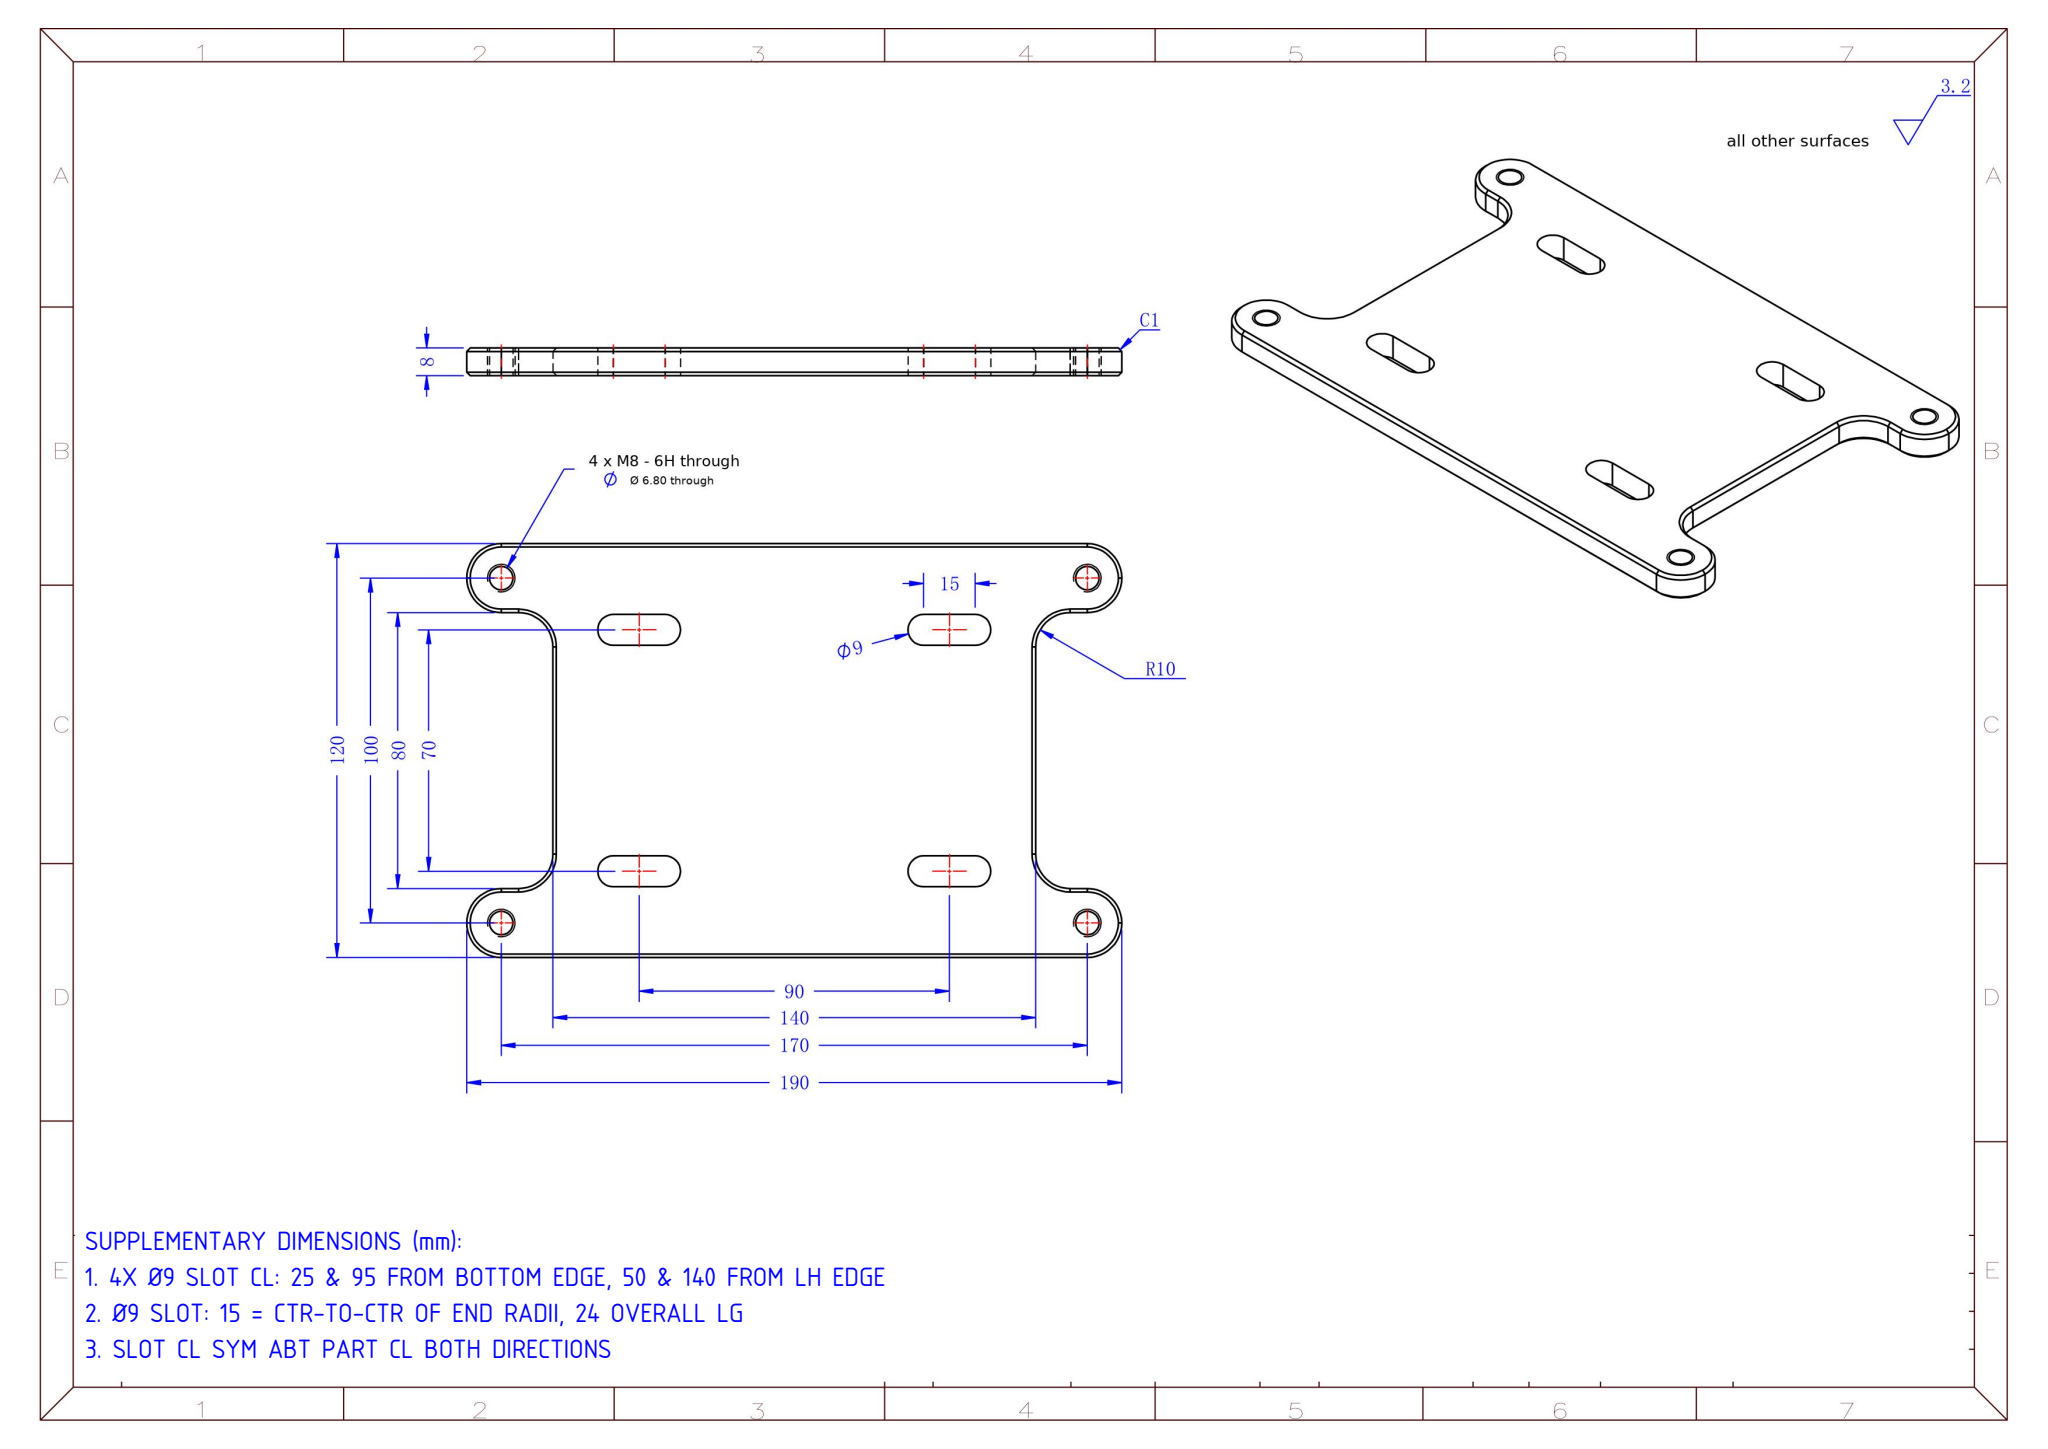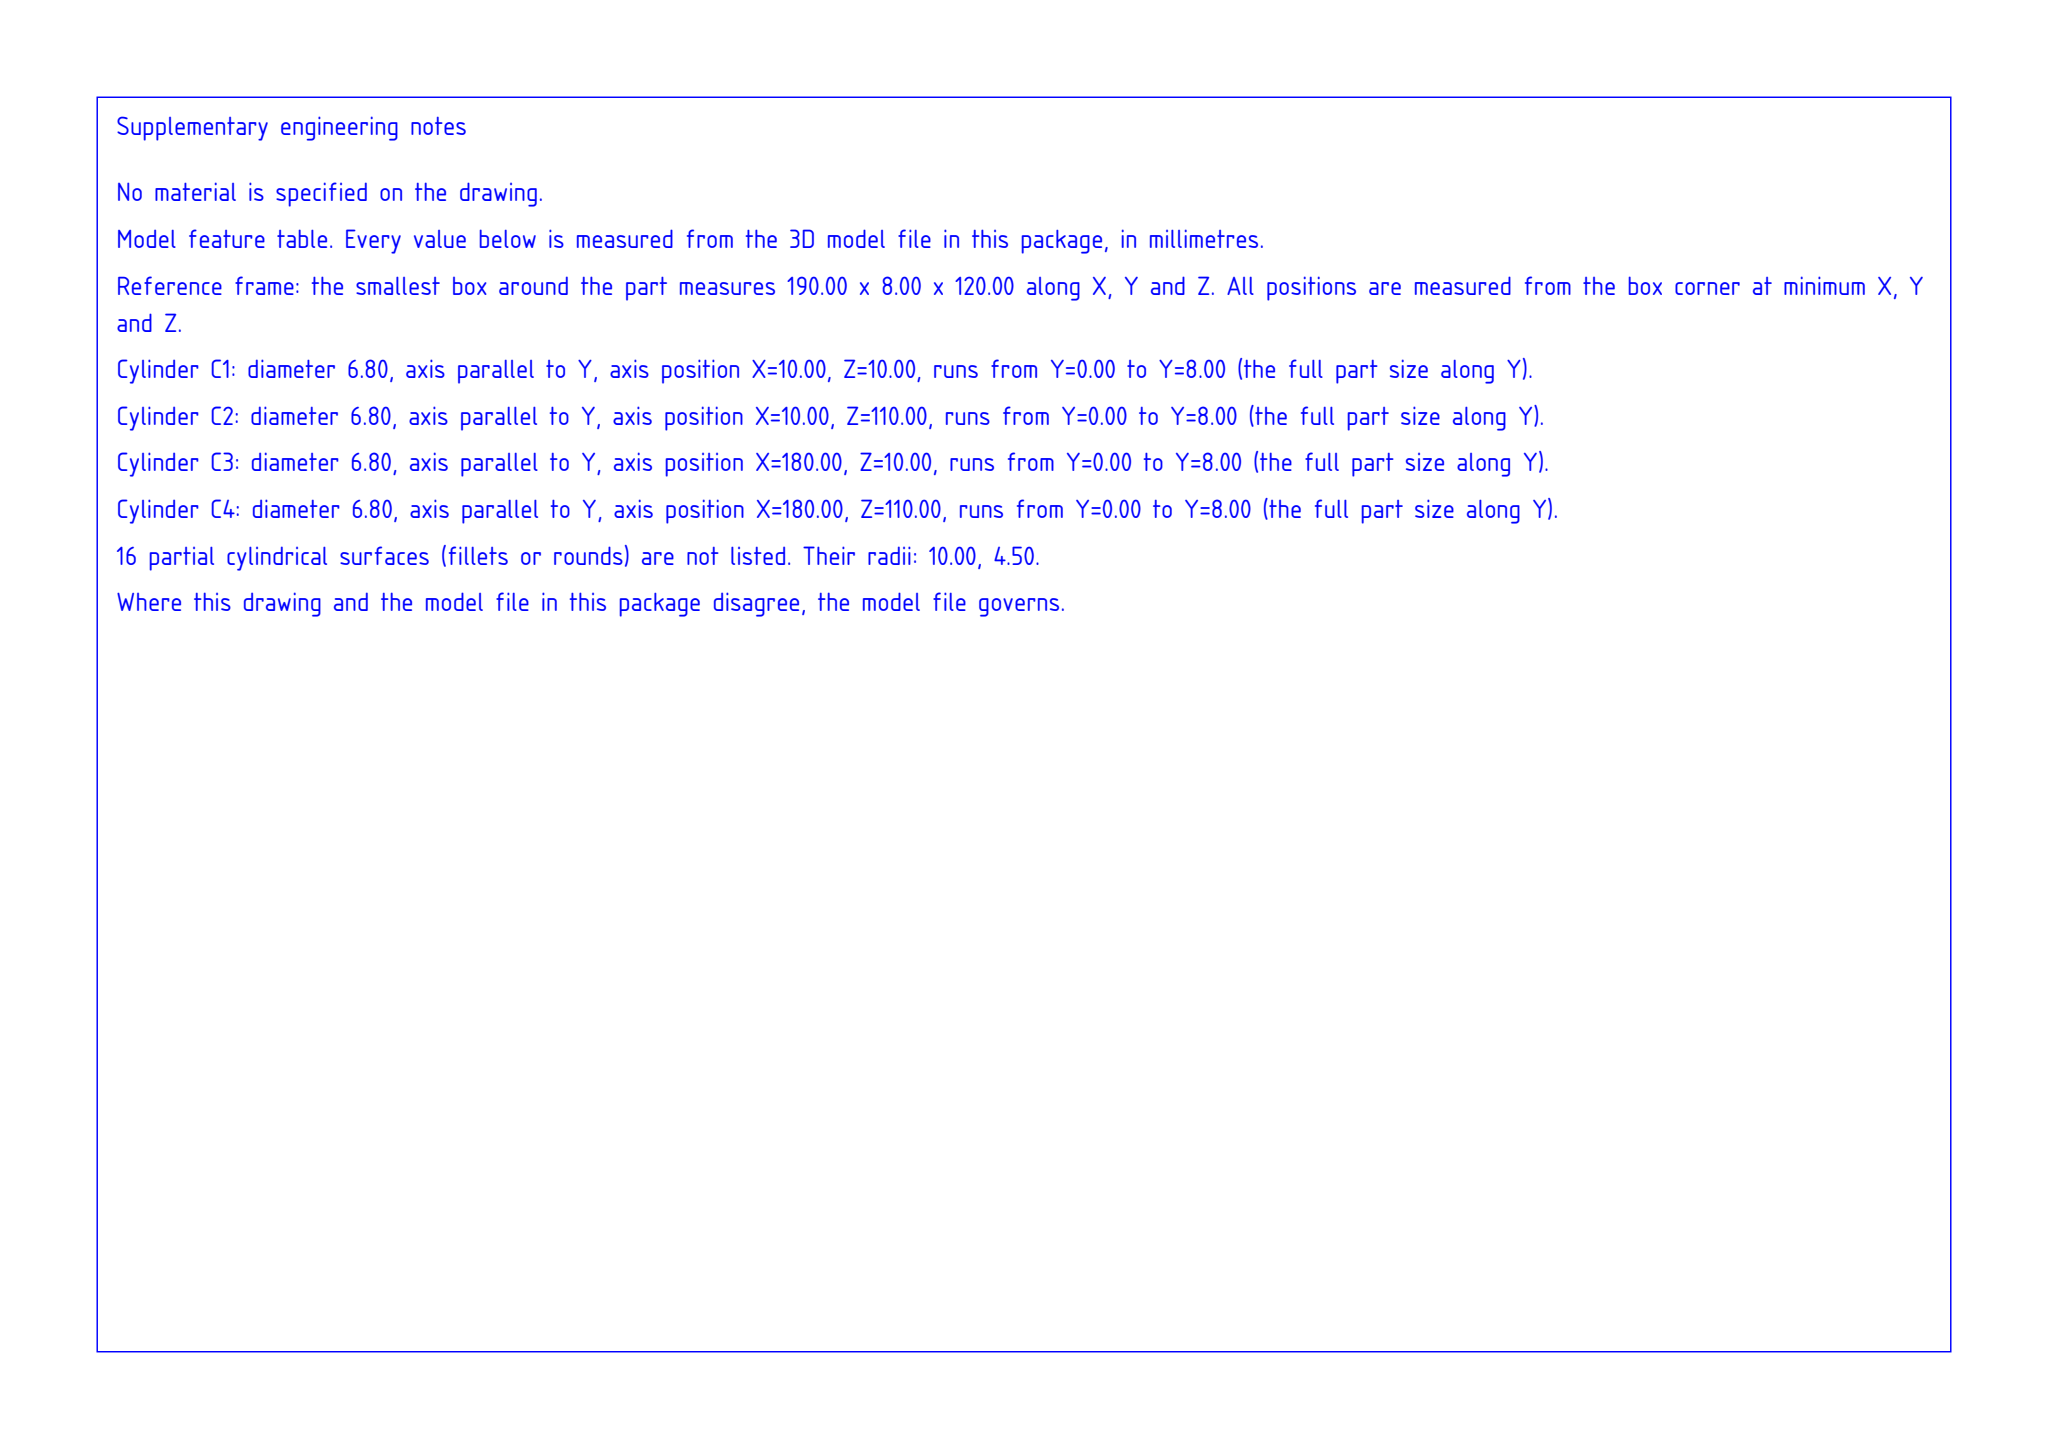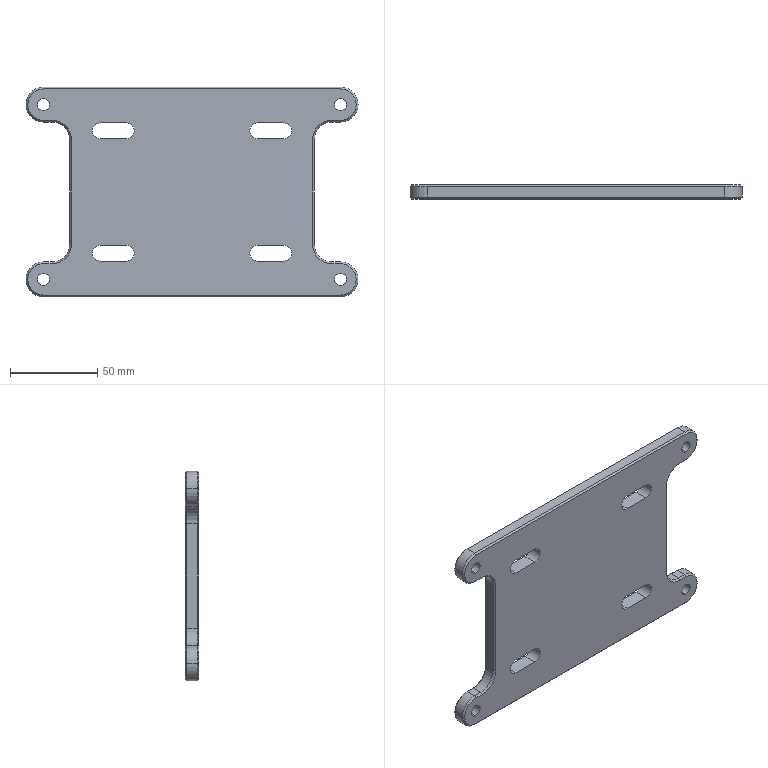Part | SolidWorks | mm | 1 solid | 86 faces | box 190 x 8 x 120 mm | volume 141529 mm3 | plane 34 | cylinder 28 | cone 24 | commonest cylinder face diameters 20 x12 6.8 x8 9 x8